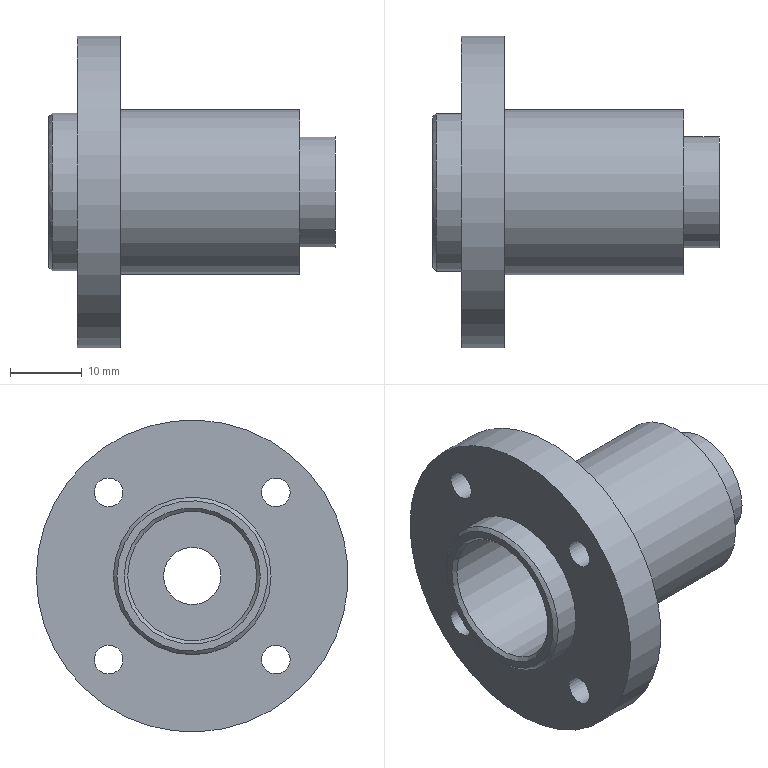Component | NX | CLHKJG_09_CYLINDER_SUPPORT | 1 solid | 18 faces | volume 13518 mm3 | cylinder 10 | plane 6 | cone 2 | commonest cylinder face diameters 4 x4 43.5 x1 22 x1 23 x1 15.5 x1 18 x1 8 x1